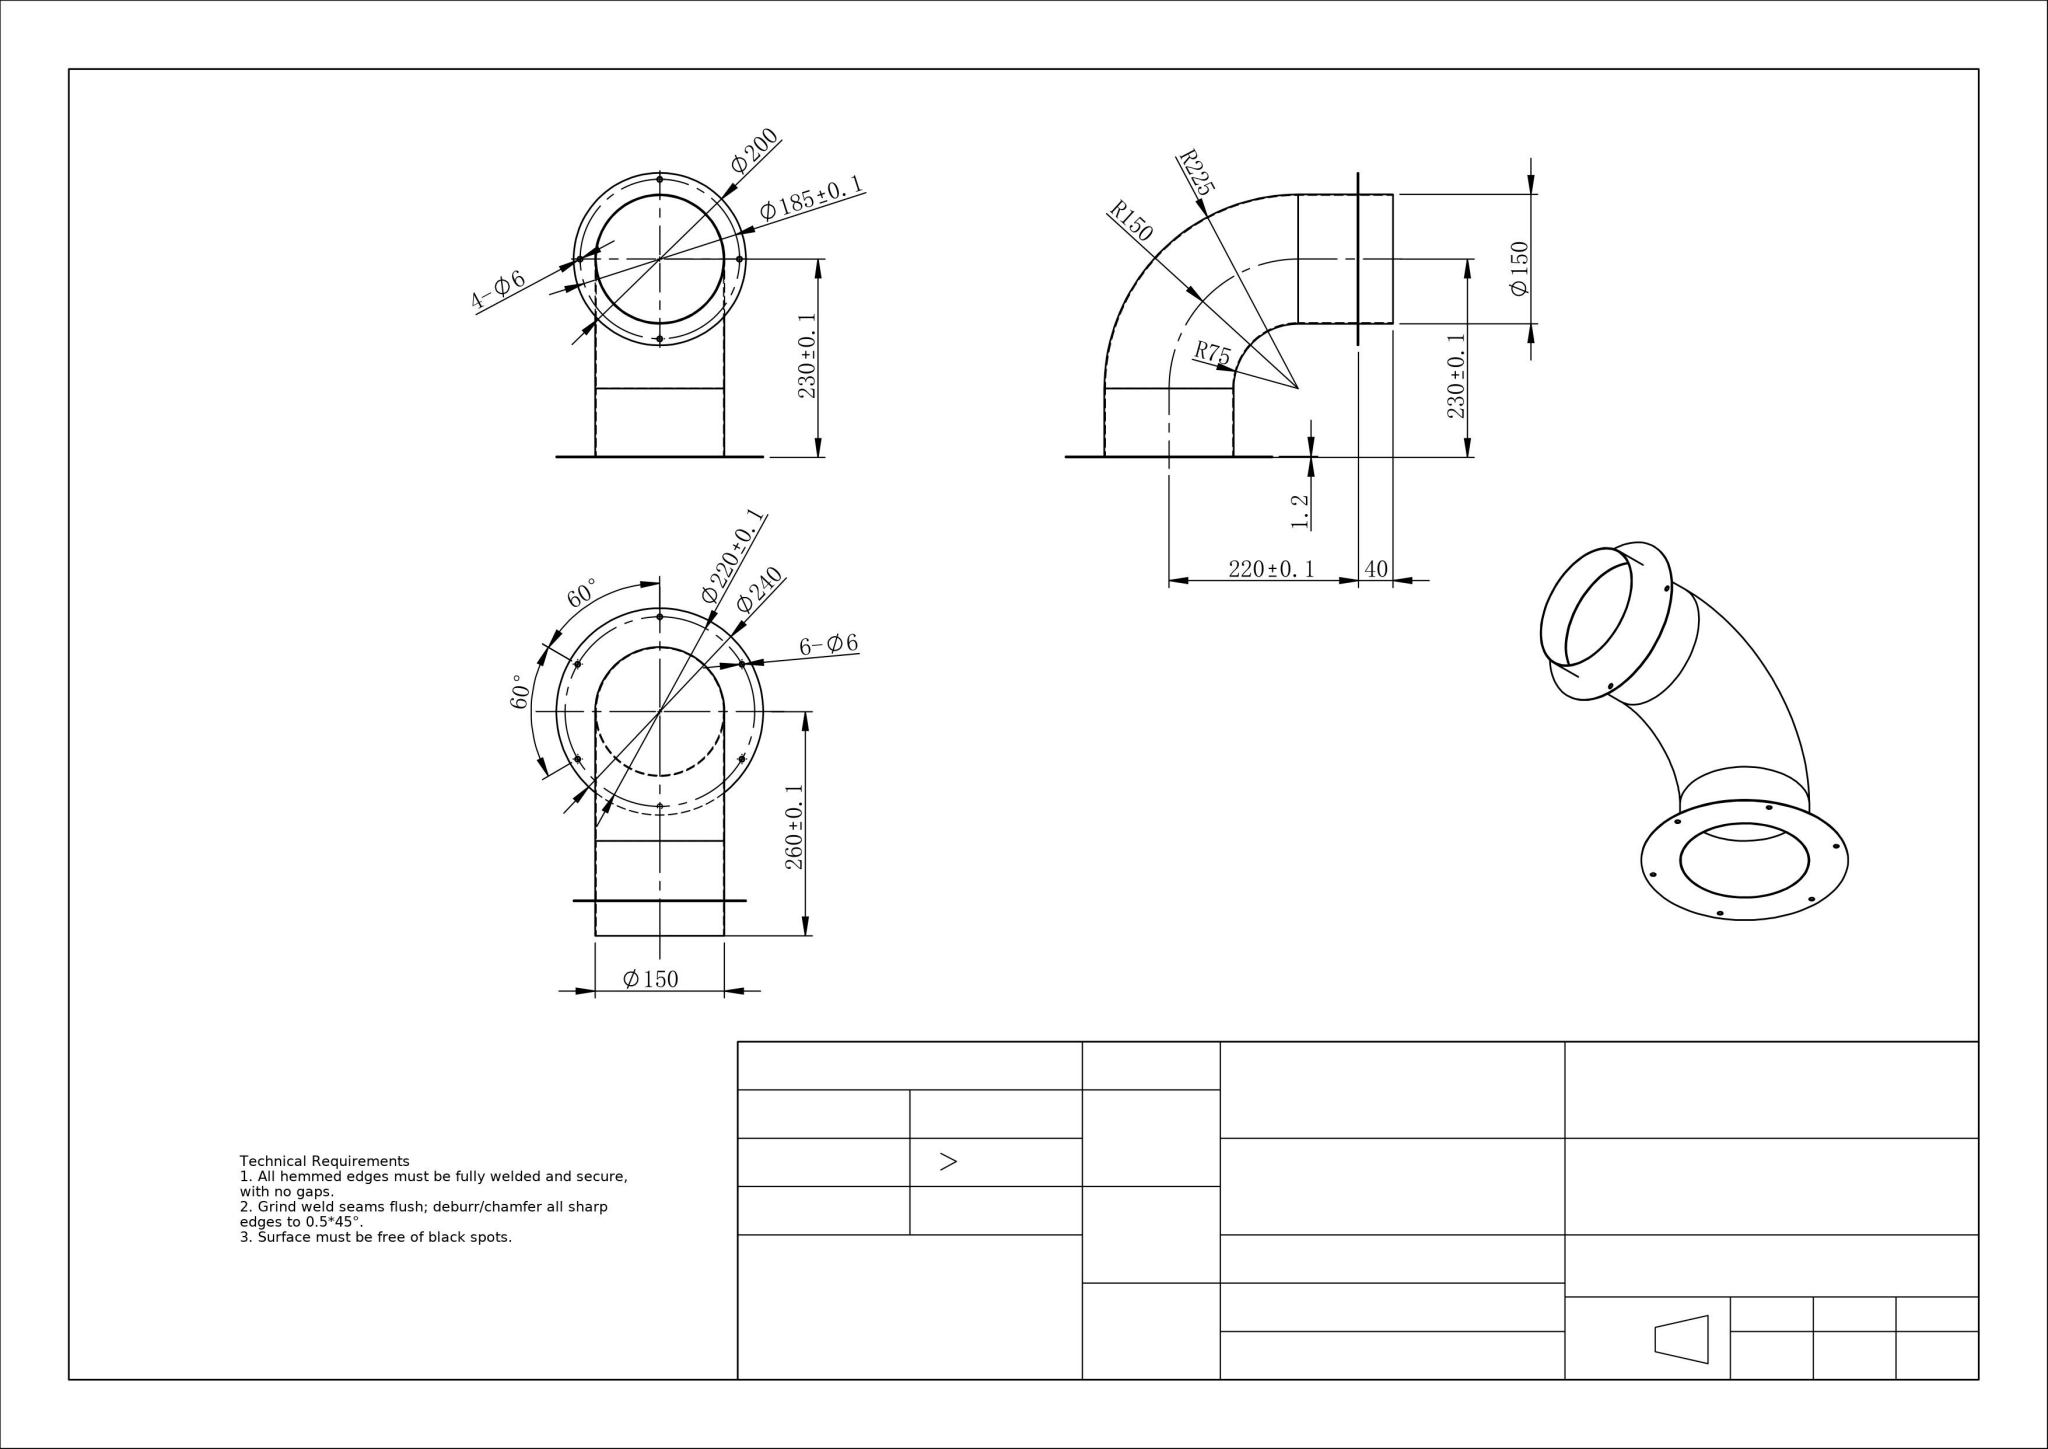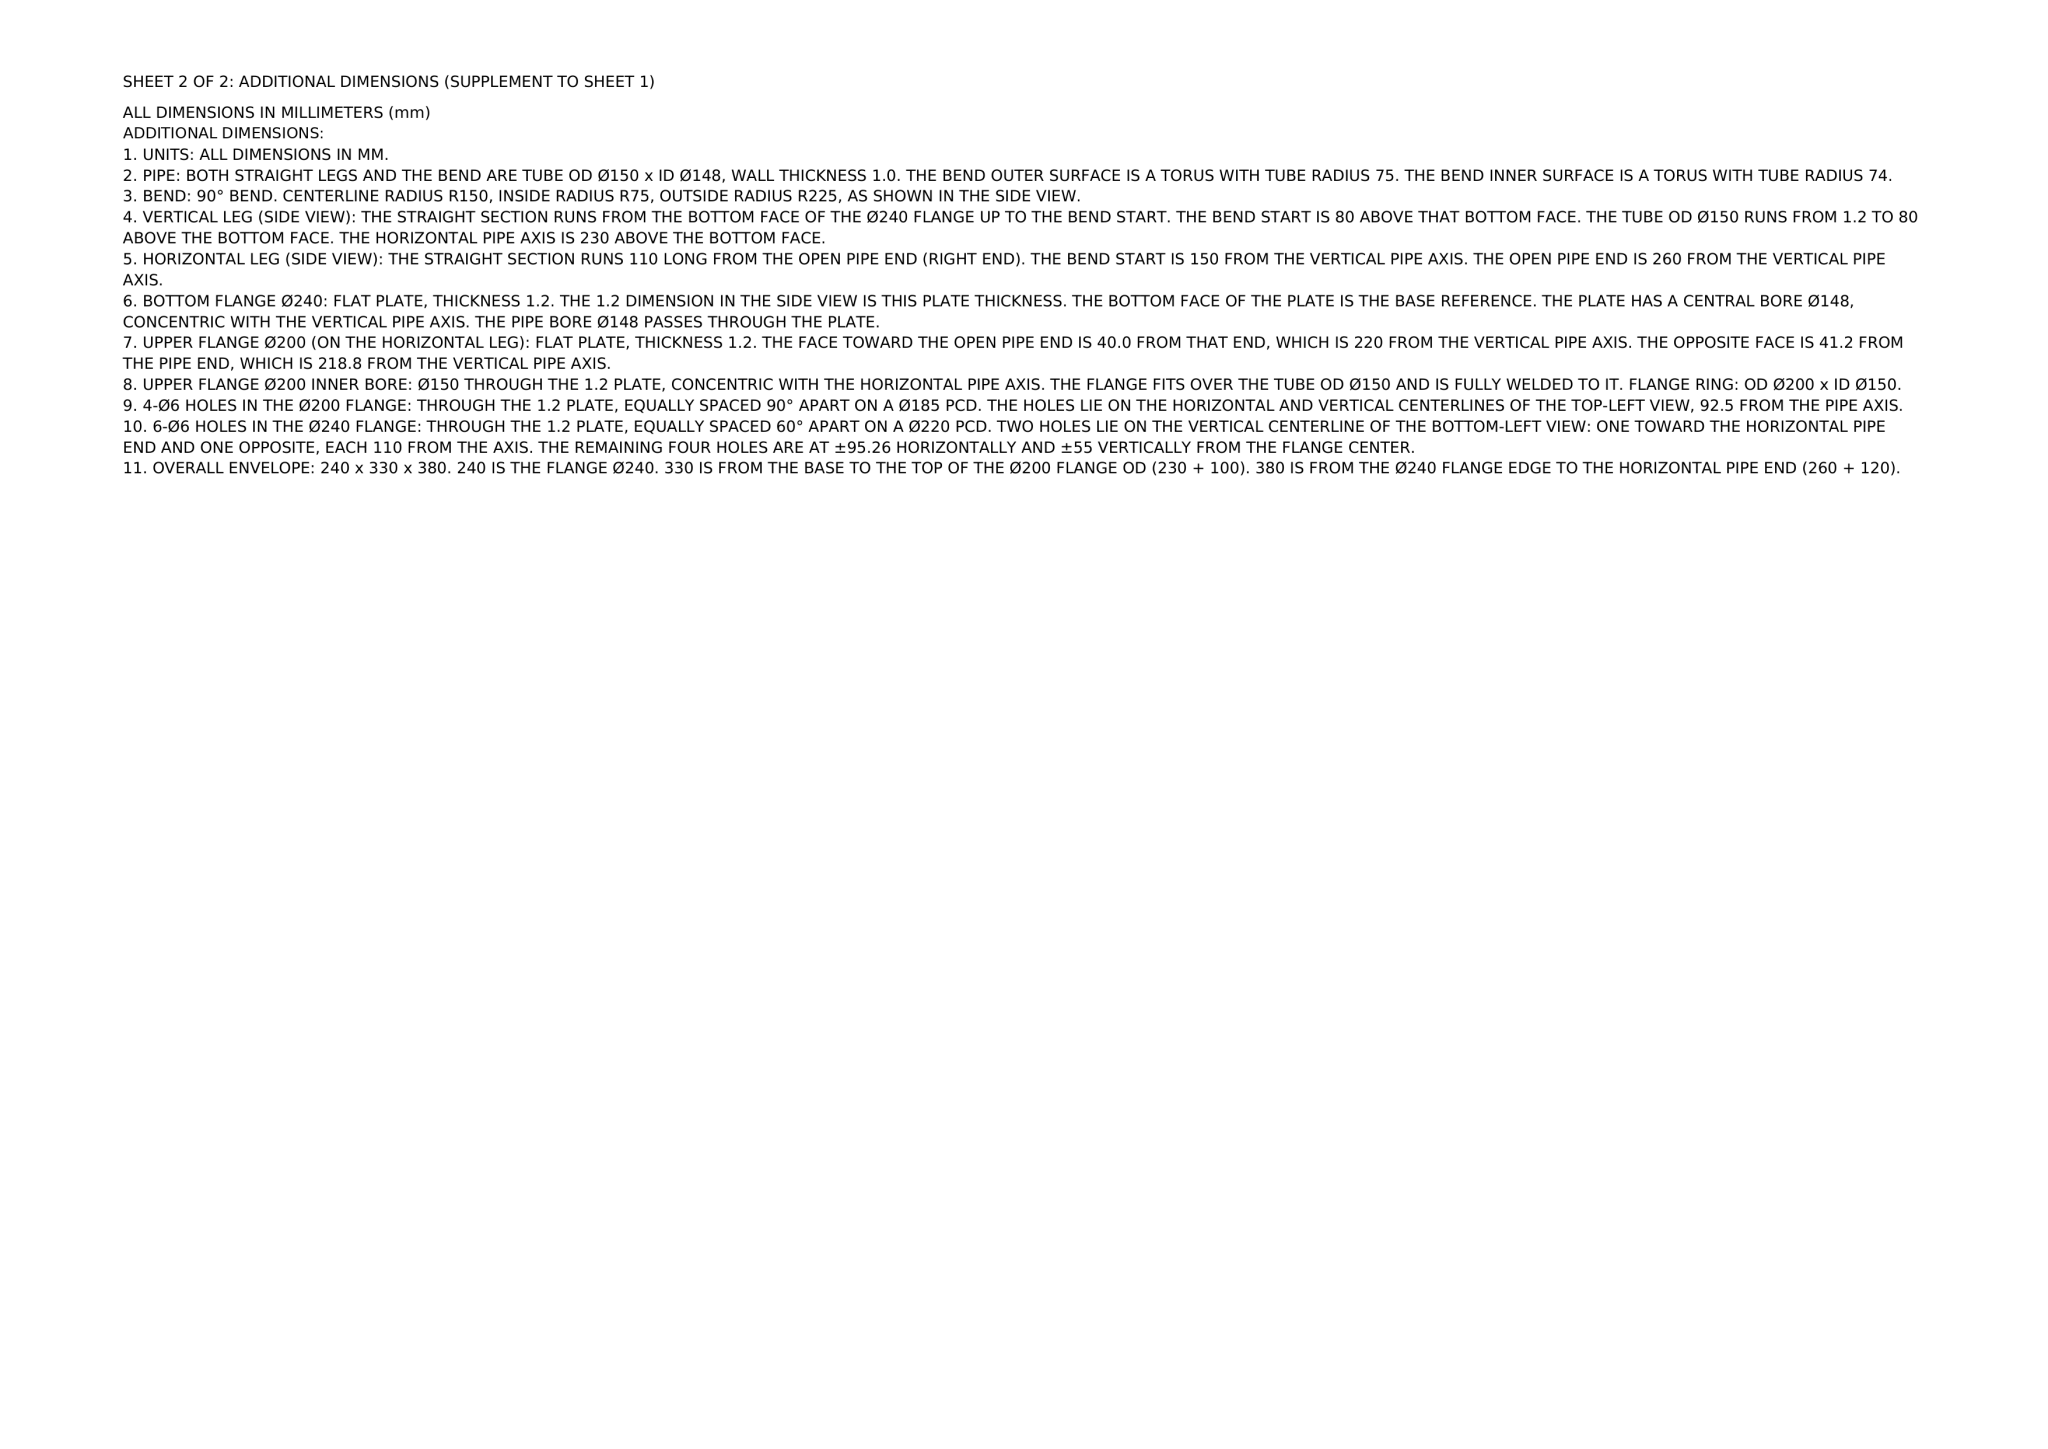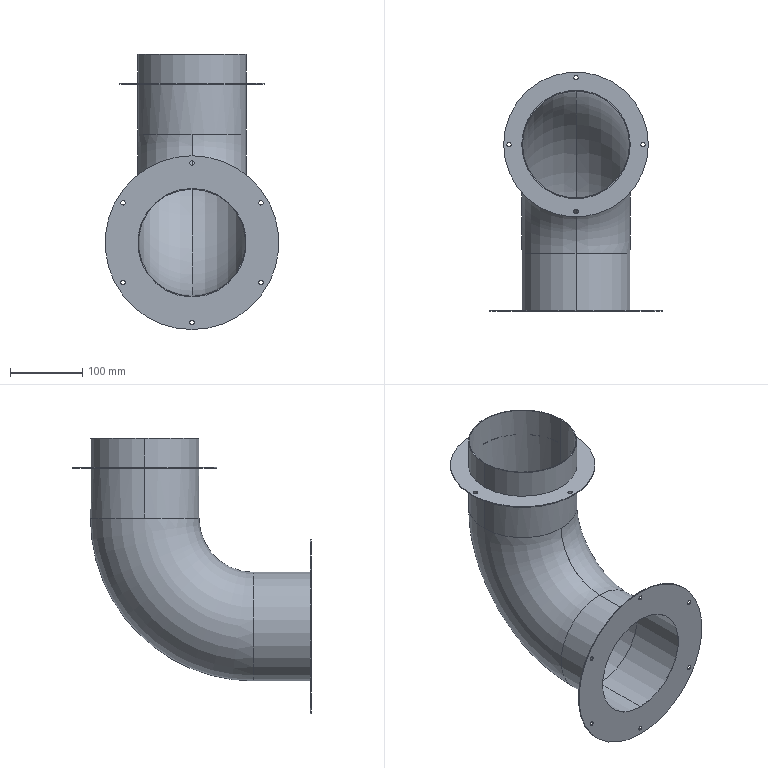Part | NX | mm | 1 solid | 43 faces | box 240 x 330 x 380 mm | volume 248466 mm3 | cylinder 34 | plane 5 | torus 4 | commonest cylinder face diameters 6 x20 150 x6 148 x4 240 x2 200 x2